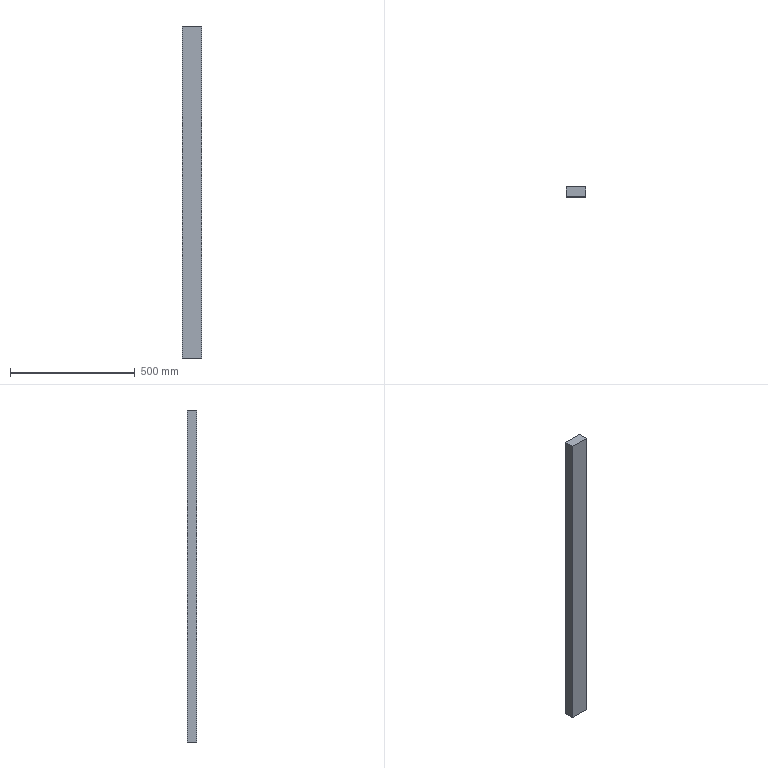Component | SolidWorks | 40x40X607Profile-1 | 1 solid | 6 faces | box 80 x 40 x 1330 mm | volume 4256000 mm3 | plane 6 | material Plain Carbon Steel
build123d program:
from build123d import *

# Parameters (mm, degrees)
SKETCH1_W           = 80
SKETCH1_H           = 40
BOSS_EXTRUDE1_DEPTH = 1330


with BuildPart() as part:
    # Sketch1 → Boss-Extrude1 (new body)
    with BuildSketch(Plane.XY):
        with Locations((0.007312, 0)):
            Rectangle(SKETCH1_W, SKETCH1_H)
    extrude(amount=BOSS_EXTRUDE1_DEPTH)


solid = part.part

# Placed as in the assembly
solid = solid.moved(Location((-4.557, 5.646, 180), (0, 0, 0)))
STEP:
#1=COLOUR_RGB('',0.7922,0.8196,0.9333);
#2=FILL_AREA_STYLE_COLOUR('',#1);
#3=FILL_AREA_STYLE('',(#2));
#4=SURFACE_STYLE_FILL_AREA(#3);
#5=SURFACE_SIDE_STYLE('',(#4));
#6=SURFACE_STYLE_USAGE(.BOTH.,#5);
#7=PRESENTATION_STYLE_ASSIGNMENT((#6));
#8=CARTESIAN_POINT('',(1.396,1.01,7.087));
#9=VERTEX_POINT('',#8);
#10=CARTESIAN_POINT('',(-1.754,1.01,7.087));
#11=VERTEX_POINT('',#10);
#12=CARTESIAN_POINT('',(1.396,1.01,7.087));
#13=DIRECTION('',(-1.,-0.,0.));
#14=VECTOR('',#13,39.37);
#15=LINE('',#12,#14);
#16=EDGE_CURVE('',#9,#11,#15,.T.);
#17=ORIENTED_EDGE('',*,*,#16,.T.);
#18=CARTESIAN_POINT('',(-1.754,1.01,59.449));
#19=VERTEX_POINT('',#18);
#20=CARTESIAN_POINT('',(-1.754,1.01,59.449));
#21=DIRECTION('',(0.,0.,-1.));
#22=VECTOR('',#21,39.37);
#23=LINE('',#20,#22);
#24=EDGE_CURVE('',#19,#11,#23,.T.);
#25=ORIENTED_EDGE('',*,*,#24,.F.);
#26=CARTESIAN_POINT('',(1.396,1.01,59.449));
#27=VERTEX_POINT('',#26);
#28=CARTESIAN_POINT('',(1.396,1.01,59.449));
#29=DIRECTION('',(-1.,-0.,0.));
#30=VECTOR('',#29,39.37);
#31=LINE('',#28,#30);
#32=EDGE_CURVE('',#27,#19,#31,.T.);
#33=ORIENTED_EDGE('',*,*,#32,.F.);
#34=CARTESIAN_POINT('',(1.396,1.01,59.449));
#35=DIRECTION('',(0.,0.,-1.));
#36=VECTOR('',#35,39.37);
#37=LINE('',#34,#36);
#38=EDGE_CURVE('',#27,#9,#37,.T.);
#39=ORIENTED_EDGE('',*,*,#38,.T.);
#40=EDGE_LOOP('',(#17,#25,#33,#39));
#41=FACE_OUTER_BOUND('',#40,.T.);
#42=CARTESIAN_POINT('',(1.396,1.01,59.449));
#43=DIRECTION('',(0.,-1.,0.));
#44=DIRECTION('',(1.,0.,0.));
#45=AXIS2_PLACEMENT_3D('',#42,#43,#44);
#46=PLANE('',#45);
#47=ADVANCED_FACE('',(#41),#46,.F.);
#48=CARTESIAN_POINT('',(-1.754,-0.5651,7.087));
#49=VERTEX_POINT('',#48);
#50=CARTESIAN_POINT('',(-1.754,-0.5651,7.087));
#51=DIRECTION('',(0.,-1.,0.));
#52=VECTOR('',#51,39.37);
#53=LINE('',#50,#52);
#54=EDGE_CURVE('',#11,#49,#53,.T.);
#55=ORIENTED_EDGE('',*,*,#54,.T.);
#56=CARTESIAN_POINT('',(-1.754,-0.5651,59.449));
#57=VERTEX_POINT('',#56);
#58=CARTESIAN_POINT('',(-1.754,-0.5651,59.449));
#59=DIRECTION('',(0.,0.,-1.));
#60=VECTOR('',#59,39.37);
#61=LINE('',#58,#60);
#62=EDGE_CURVE('',#57,#49,#61,.T.);
#63=ORIENTED_EDGE('',*,*,#62,.F.);
#64=CARTESIAN_POINT('',(-1.754,-0.5651,59.449));
#65=DIRECTION('',(0.,-1.,0.));
#66=VECTOR('',#65,39.37);
#67=LINE('',#64,#66);
#68=EDGE_CURVE('',#19,#57,#67,.T.);
#69=ORIENTED_EDGE('',*,*,#68,.F.);
#70=ORIENTED_EDGE('',*,*,#24,.T.);
#71=EDGE_LOOP('',(#55,#63,#69,#70));
#72=FACE_OUTER_BOUND('',#71,.T.);
#73=CARTESIAN_POINT('',(-1.754,-0.5651,59.449));
#74=DIRECTION('',(1.,0.,0.));
#75=DIRECTION('',(0.,0.,-1.));
#76=AXIS2_PLACEMENT_3D('',#73,#74,#75);
#77=PLANE('',#76);
#78=ADVANCED_FACE('',(#72),#77,.F.);
#79=CARTESIAN_POINT('',(1.396,-0.5651,7.087));
#80=VERTEX_POINT('',#79);
#81=CARTESIAN_POINT('',(1.396,-0.5651,7.087));
#82=DIRECTION('',(1.,0.,0.));
#83=VECTOR('',#82,39.37);
#84=LINE('',#81,#83);
#85=EDGE_CURVE('',#49,#80,#84,.T.);
#86=ORIENTED_EDGE('',*,*,#85,.T.);
#87=CARTESIAN_POINT('',(1.396,-0.5651,59.449));
#88=VERTEX_POINT('',#87);
#89=CARTESIAN_POINT('',(1.396,-0.5651,59.449));
#90=DIRECTION('',(0.,0.,-1.));
#91=VECTOR('',#90,39.37);
#92=LINE('',#89,#91);
#93=EDGE_CURVE('',#88,#80,#92,.T.);
#94=ORIENTED_EDGE('',*,*,#93,.F.);
#95=CARTESIAN_POINT('',(1.396,-0.5651,59.449));
#96=DIRECTION('',(1.,0.,0.));
#97=VECTOR('',#96,39.37);
#98=LINE('',#95,#97);
#99=EDGE_CURVE('',#57,#88,#98,.T.);
#100=ORIENTED_EDGE('',*,*,#99,.F.);
#101=ORIENTED_EDGE('',*,*,#62,.T.);
#102=EDGE_LOOP('',(#86,#94,#100,#101));
#103=FACE_OUTER_BOUND('',#102,.T.);
#104=CARTESIAN_POINT('',(1.396,-0.5651,59.449));
#105=DIRECTION('',(-0.,1.,0.));
#106=DIRECTION('',(-1.,-0.,0.));
#107=AXIS2_PLACEMENT_3D('',#104,#105,#106);
#108=PLANE('',#107);
#109=ADVANCED_FACE('',(#103),#108,.F.);
#110=CARTESIAN_POINT('',(1.396,-0.5651,7.087));
#111=DIRECTION('',(0.,1.,0.));
#112=VECTOR('',#111,39.37);
#113=LINE('',#110,#112);
#114=EDGE_CURVE('',#80,#9,#113,.T.);
#115=ORIENTED_EDGE('',*,*,#114,.T.);
#116=ORIENTED_EDGE('',*,*,#38,.F.);
#117=CARTESIAN_POINT('',(1.396,-0.5651,59.449));
#118=DIRECTION('',(0.,1.,0.));
#119=VECTOR('',#118,39.37);
#120=LINE('',#117,#119);
#121=EDGE_CURVE('',#88,#27,#120,.T.);
#122=ORIENTED_EDGE('',*,*,#121,.F.);
#123=ORIENTED_EDGE('',*,*,#93,.T.);
#124=EDGE_LOOP('',(#115,#116,#122,#123));
#125=FACE_OUTER_BOUND('',#124,.T.);
#126=CARTESIAN_POINT('',(1.396,-0.5651,59.449));
#127=DIRECTION('',(-1.,0.,0.));
#128=DIRECTION('',(0.,0.,1.));
#129=AXIS2_PLACEMENT_3D('',#126,#127,#128);
#130=PLANE('',#129);
#131=ADVANCED_FACE('',(#125),#130,.F.);
#132=ORIENTED_EDGE('',*,*,#32,.T.);
#133=ORIENTED_EDGE('',*,*,#68,.T.);
#134=ORIENTED_EDGE('',*,*,#99,.T.);
#135=ORIENTED_EDGE('',*,*,#121,.T.);
#136=EDGE_LOOP('',(#132,#133,#134,#135));
#137=FACE_OUTER_BOUND('',#136,.T.);
#138=CARTESIAN_POINT('',(-0.1794,0.2223,59.449));
#139=DIRECTION('',(0.,0.,-1.));
#140=DIRECTION('',(-1.,0.,0.));
#141=AXIS2_PLACEMENT_3D('',#138,#139,#140);
#142=PLANE('',#141);
#143=ADVANCED_FACE('',(#137),#142,.F.);
#144=ORIENTED_EDGE('',*,*,#16,.F.);
#145=ORIENTED_EDGE('',*,*,#114,.F.);
#146=ORIENTED_EDGE('',*,*,#85,.F.);
#147=ORIENTED_EDGE('',*,*,#54,.F.);
#148=EDGE_LOOP('',(#144,#145,#146,#147));
#149=FACE_OUTER_BOUND('',#148,.T.);
#150=CARTESIAN_POINT('',(-0.1794,0.2223,7.087));
#151=DIRECTION('',(0.,0.,-1.));
#152=DIRECTION('',(-1.,0.,0.));
#153=AXIS2_PLACEMENT_3D('',#150,#151,#152);
#154=PLANE('',#153);
#155=ADVANCED_FACE('',(#149),#154,.T.);
#156=CLOSED_SHELL('',(#47,#78,#109,#131,#143,#155));
#157=MANIFOLD_SOLID_BREP('',#156);
#158=STYLED_ITEM('',(#7),#157);
#159=(LENGTH_UNIT()NAMED_UNIT(*)SI_UNIT($,.METRE.));
#160=LENGTH_MEASURE_WITH_UNIT(LENGTH_MEASURE(0.0254),#159);
#161=DIMENSIONAL_EXPONENTS(1.,0.,0.,0.,0.,0.,0.);
#162=(CONVERSION_BASED_UNIT('',#160)LENGTH_UNIT()NAMED_UNIT(#161));
#163=UNCERTAINTY_MEASURE_WITH_UNIT(LENGTH_MEASURE(0.00001),#162,'','');
#164=(NAMED_UNIT(*)PLANE_ANGLE_UNIT()SI_UNIT($,.RADIAN.));
#165=(NAMED_UNIT(*)SI_UNIT($,.STERADIAN.)SOLID_ANGLE_UNIT());
#166=(GEOMETRIC_REPRESENTATION_CONTEXT(3)GLOBAL_UNCERTAINTY_ASSIGNED_CONTEXT((#163))GLOBAL_UNIT_ASSIGNED_CONTEXT((#162,#164,#165))REPRESENTATION_CONTEXT('',''));
#167=MECHANICAL_DESIGN_GEOMETRIC_PRESENTATION_REPRESENTATION('',(#158),#166);
#168=PRESENTATION_LAYER_ASSIGNMENT('','',(#158));
#169=CARTESIAN_POINT('',(0.,0.,0.));
#170=DIRECTION('',(0.,0.,1.));
#171=DIRECTION('',(1.,0.,0.));
#172=AXIS2_PLACEMENT_3D('',#169,#170,#171);
#173=(LENGTH_UNIT()NAMED_UNIT(*)SI_UNIT($,.METRE.));
#174=LENGTH_MEASURE_WITH_UNIT(LENGTH_MEASURE(0.0254),#173);
#175=DIMENSIONAL_EXPONENTS(1.,0.,0.,0.,0.,0.,0.);
#176=(CONVERSION_BASED_UNIT('',#174)LENGTH_UNIT()NAMED_UNIT(#175));
#177=UNCERTAINTY_MEASURE_WITH_UNIT(LENGTH_MEASURE(0.00001),#176,'','');
#178=(NAMED_UNIT(*)PLANE_ANGLE_UNIT()SI_UNIT($,.RADIAN.));
#179=(NAMED_UNIT(*)SI_UNIT($,.STERADIAN.)SOLID_ANGLE_UNIT());
#180=(GEOMETRIC_REPRESENTATION_CONTEXT(3)GLOBAL_UNCERTAINTY_ASSIGNED_CONTEXT((#177))GLOBAL_UNIT_ASSIGNED_CONTEXT((#176,#178,#179))REPRESENTATION_CONTEXT('',''));
#181=ADVANCED_BREP_SHAPE_REPRESENTATION('',(#157,#172),#180);